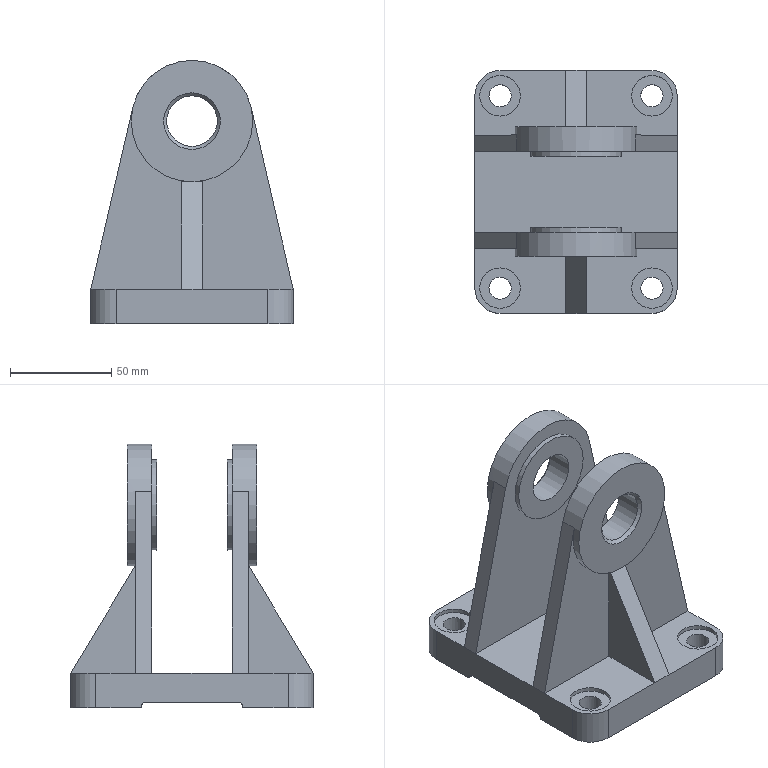Component | NX | 5 | 1 solid | 60 faces | volume 344259 mm3 | plane 38 | cylinder 20 | cone 2 | commonest cylinder face diameters 25 x6 11 x4 20 x4 60 x2 45 x2 4 x2